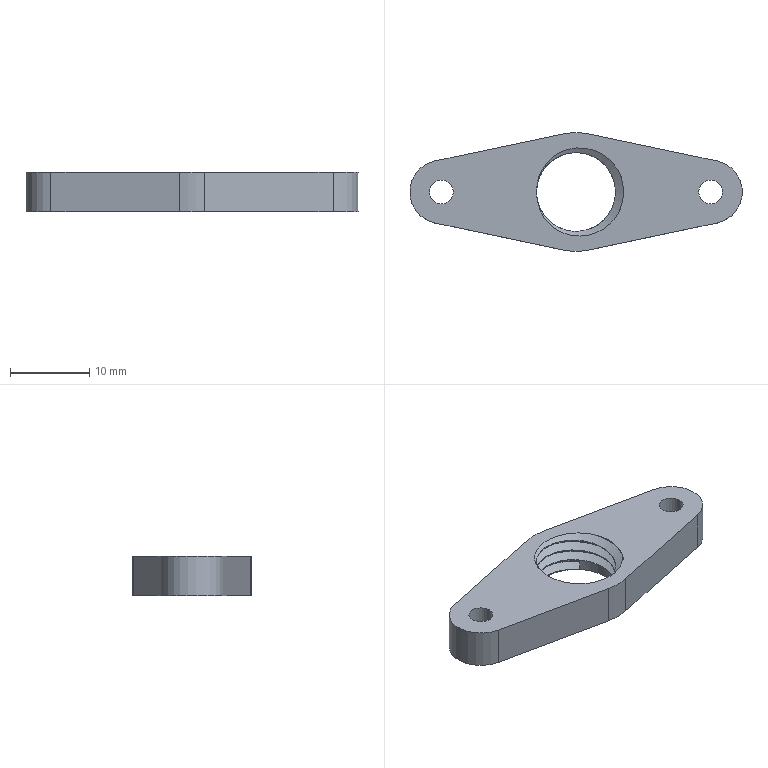Component | NX | FASTENER | 1 solid | 17 faces | volume 1706 mm3 | cylinder 8 | plane 7 | spline 2 | commonest cylinder face diameters 15 x2 8 x2 3 x2 10 x1 12 x1